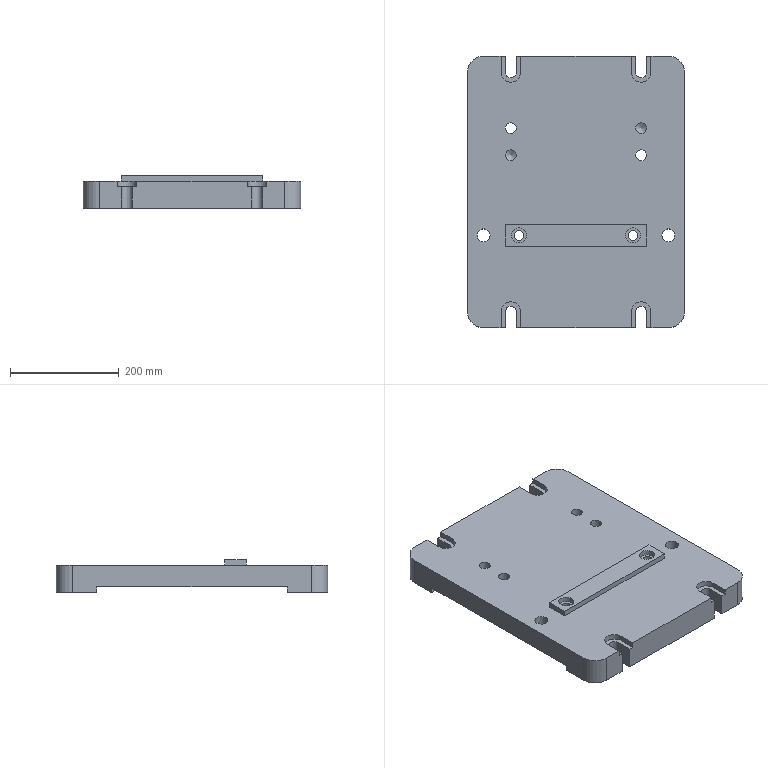Component | NX | FIXTURE_BODY | 1 solid | 65 faces | volume 8366577 mm3 | plane 41 | cylinder 22 | cone 2 | commonest cylinder face diameters 20 x8 36 x4 60 x4 24 x2 18 x2 28 x2